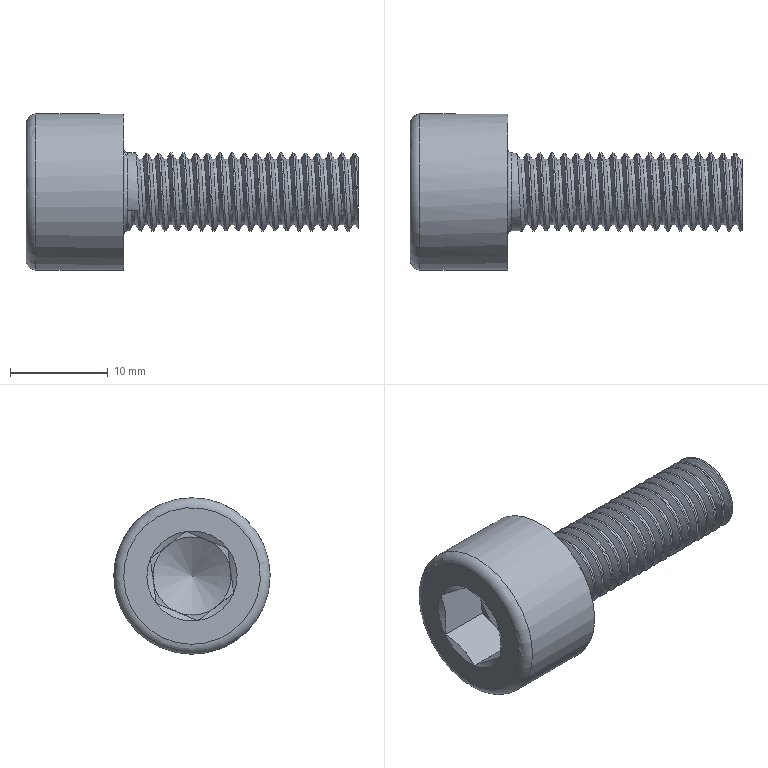Component | NX | M8X24_HEX_BOLT_2 | 1 solid | 30 faces | volume 2700 mm3 | plane 16 | cone 7 | cylinder 3 | torus 2 | spline 2 | commonest cylinder face diameters 8 x1 16 x1 6.75 x1